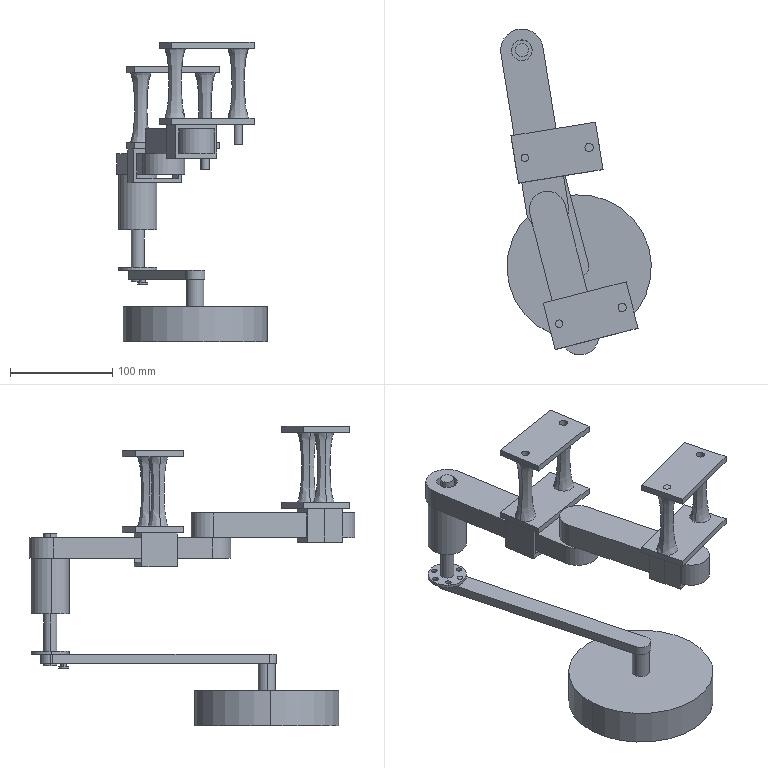Component | SolidWorks | MirrorJoint-2 | 19 solids | 179 faces | volume 1105530 mm3 | cylinder 86 | plane 85 | spline 8 | commonest cylinder face diameters 7.212 x17 8.088 x16 5.358 x16 12.936 x8 37.268 x4 20.14 x4 18.491 x4 16.846 x4